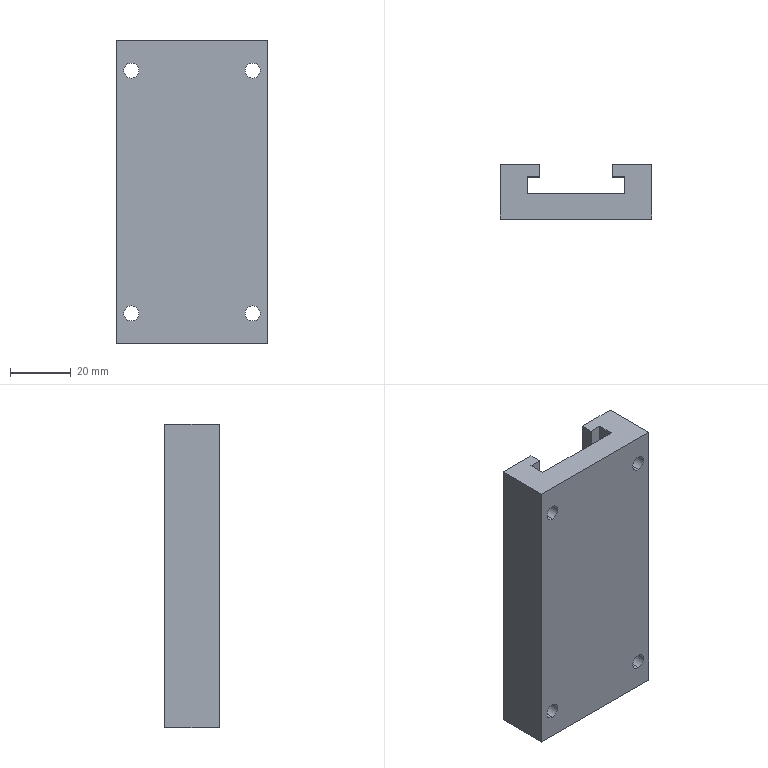Component | SolidWorks | 8TC-A15004-D0-13A-2 | 1 solid | 22 faces | box 50 x 18 x 100 mm | volume 61386 mm3 | plane 14 | cylinder 8 | commonest cylinder face diameters 5 x8 | material #45
build123d program:
from build123d import *

# Parameters (mm, degrees)
SKETCH1_W           = 100
SKETCH1_H           = 50
BOSS_EXTRUDE1_DEPTH = 18
CUT_EXTRUDE1_DEPTH  = 105.637
M6_TAPPED_HOLE1_D   = 5


with BuildPart() as part:
    # Sketch1 → Boss-Extrude1 (new body)
    with BuildSketch(Plane.XY):
        Rectangle(SKETCH1_W, SKETCH1_H)
    extrude(amount=BOSS_EXTRUDE1_DEPTH)

    # Sketch2 → Cut-Extrude1 (cut, through all)
    with BuildSketch(Plane(origin=(50, 0, 0), x_dir=(0, 0, -1), z_dir=(1, 0, 0))):
        Polygon((-8.5, -16), (-8.5, 16), (-14, 16), (-14, 12), (-18, 12), (-18, -12), (-14, -12), (-14, -16), align=None)
    extrude(amount=-CUT_EXTRUDE1_DEPTH, mode=Mode.SUBTRACT)

    # M6 Tapped Hole1 (through all)
    with Locations(Plane(origin=(0, 0, 0), x_dir=(-1, 0, 0), z_dir=(0, 0, -1))):
        with Locations((-40, 20), (-40, -20), (40, -20), (40, 20)):
            Hole(M6_TAPPED_HOLE1_D / 2)


solid = part.part

# Placed as in the assembly
solid = solid.moved(Location((-7.5, 344.5, 0), (-90, 0, 90)))
STEP:
#1=COLOUR_RGB('',0.7922,0.8196,0.9333);
#2=FILL_AREA_STYLE_COLOUR('',#1);
#3=FILL_AREA_STYLE('',(#2));
#4=SURFACE_STYLE_FILL_AREA(#3);
#5=SURFACE_SIDE_STYLE('',(#4));
#6=SURFACE_STYLE_USAGE(.BOTH.,#5);
#7=PRESENTATION_STYLE_ASSIGNMENT((#6));
#8=CARTESIAN_POINT('',(-1.083,14.272,-1.673));
#9=VERTEX_POINT('',#8);
#10=CARTESIAN_POINT('',(-1.083,14.272,-1.476));
#11=VERTEX_POINT('',#10);
#12=CARTESIAN_POINT('',(-1.083,14.272,-1.575));
#13=DIRECTION('',(0.,-1.,-0.));
#14=DIRECTION('',(0.,0.,1.));
#15=AXIS2_PLACEMENT_3D('',#12,#13,#14);
#16=CIRCLE('',#15,0.09843);
#17=EDGE_CURVE('',#9,#11,#16,.T.);
#18=ORIENTED_EDGE('',*,*,#17,.F.);
#19=CARTESIAN_POINT('',(-1.083,13.563,-1.673));
#20=VERTEX_POINT('',#19);
#21=CARTESIAN_POINT('',(-1.083,13.563,-1.673));
#22=DIRECTION('',(0.,-1.,-0.));
#23=VECTOR('',#22,39.37);
#24=LINE('',#21,#23);
#25=EDGE_CURVE('',#9,#20,#24,.T.);
#26=ORIENTED_EDGE('',*,*,#25,.T.);
#27=CARTESIAN_POINT('',(-1.083,13.563,-1.476));
#28=VERTEX_POINT('',#27);
#29=CARTESIAN_POINT('',(-1.083,13.563,-1.575));
#30=DIRECTION('',(0.,-1.,-0.));
#31=DIRECTION('',(0.,0.,1.));
#32=AXIS2_PLACEMENT_3D('',#29,#30,#31);
#33=CIRCLE('',#32,0.09843);
#34=EDGE_CURVE('',#20,#28,#33,.T.);
#35=ORIENTED_EDGE('',*,*,#34,.T.);
#36=CARTESIAN_POINT('',(-1.083,13.563,-1.476));
#37=DIRECTION('',(0.,-1.,-0.));
#38=VECTOR('',#37,39.37);
#39=LINE('',#36,#38);
#40=EDGE_CURVE('',#11,#28,#39,.T.);
#41=ORIENTED_EDGE('',*,*,#40,.F.);
#42=EDGE_LOOP('',(#18,#26,#35,#41));
#43=FACE_OUTER_BOUND('',#42,.T.);
#44=CARTESIAN_POINT('',(-1.083,13.563,-1.575));
#45=DIRECTION('',(0.,-1.,-0.));
#46=DIRECTION('',(0.,0.,1.));
#47=AXIS2_PLACEMENT_3D('',#44,#45,#46);
#48=CYLINDRICAL_SURFACE('',#47,0.09843);
#49=ADVANCED_FACE('',(#43),#48,.F.);
#50=CARTESIAN_POINT('',(0.4921,14.272,-1.673));
#51=VERTEX_POINT('',#50);
#52=CARTESIAN_POINT('',(0.4921,14.272,-1.476));
#53=VERTEX_POINT('',#52);
#54=CARTESIAN_POINT('',(0.4921,14.272,-1.575));
#55=DIRECTION('',(0.,-1.,-0.));
#56=DIRECTION('',(0.,0.,1.));
#57=AXIS2_PLACEMENT_3D('',#54,#55,#56);
#58=CIRCLE('',#57,0.09843);
#59=EDGE_CURVE('',#51,#53,#58,.T.);
#60=ORIENTED_EDGE('',*,*,#59,.F.);
#61=CARTESIAN_POINT('',(0.4921,13.563,-1.673));
#62=VERTEX_POINT('',#61);
#63=CARTESIAN_POINT('',(0.4921,13.563,-1.673));
#64=DIRECTION('',(0.,-1.,-0.));
#65=VECTOR('',#64,39.37);
#66=LINE('',#63,#65);
#67=EDGE_CURVE('',#51,#62,#66,.T.);
#68=ORIENTED_EDGE('',*,*,#67,.T.);
#69=CARTESIAN_POINT('',(0.4921,13.563,-1.476));
#70=VERTEX_POINT('',#69);
#71=CARTESIAN_POINT('',(0.4921,13.563,-1.575));
#72=DIRECTION('',(0.,-1.,-0.));
#73=DIRECTION('',(0.,0.,1.));
#74=AXIS2_PLACEMENT_3D('',#71,#72,#73);
#75=CIRCLE('',#74,0.09843);
#76=EDGE_CURVE('',#62,#70,#75,.T.);
#77=ORIENTED_EDGE('',*,*,#76,.T.);
#78=CARTESIAN_POINT('',(0.4921,13.563,-1.476));
#79=DIRECTION('',(0.,-1.,-0.));
#80=VECTOR('',#79,39.37);
#81=LINE('',#78,#80);
#82=EDGE_CURVE('',#53,#70,#81,.T.);
#83=ORIENTED_EDGE('',*,*,#82,.F.);
#84=EDGE_LOOP('',(#60,#68,#77,#83));
#85=FACE_OUTER_BOUND('',#84,.T.);
#86=CARTESIAN_POINT('',(0.4921,13.563,-1.575));
#87=DIRECTION('',(0.,-1.,-0.));
#88=DIRECTION('',(0.,0.,1.));
#89=AXIS2_PLACEMENT_3D('',#86,#87,#88);
#90=CYLINDRICAL_SURFACE('',#89,0.09843);
#91=ADVANCED_FACE('',(#85),#90,.F.);
#92=CARTESIAN_POINT('',(0.4921,14.272,1.476));
#93=VERTEX_POINT('',#92);
#94=CARTESIAN_POINT('',(0.4921,14.272,1.673));
#95=VERTEX_POINT('',#94);
#96=CARTESIAN_POINT('',(0.4921,14.272,1.575));
#97=DIRECTION('',(0.,-1.,-0.));
#98=DIRECTION('',(0.,0.,1.));
#99=AXIS2_PLACEMENT_3D('',#96,#97,#98);
#100=CIRCLE('',#99,0.09843);
#101=EDGE_CURVE('',#93,#95,#100,.T.);
#102=ORIENTED_EDGE('',*,*,#101,.F.);
#103=CARTESIAN_POINT('',(0.4921,13.563,1.476));
#104=VERTEX_POINT('',#103);
#105=CARTESIAN_POINT('',(0.4921,13.563,1.476));
#106=DIRECTION('',(0.,-1.,-0.));
#107=VECTOR('',#106,39.37);
#108=LINE('',#105,#107);
#109=EDGE_CURVE('',#93,#104,#108,.T.);
#110=ORIENTED_EDGE('',*,*,#109,.T.);
#111=CARTESIAN_POINT('',(0.4921,13.563,1.673));
#112=VERTEX_POINT('',#111);
#113=CARTESIAN_POINT('',(0.4921,13.563,1.575));
#114=DIRECTION('',(0.,-1.,-0.));
#115=DIRECTION('',(0.,0.,1.));
#116=AXIS2_PLACEMENT_3D('',#113,#114,#115);
#117=CIRCLE('',#116,0.09843);
#118=EDGE_CURVE('',#104,#112,#117,.T.);
#119=ORIENTED_EDGE('',*,*,#118,.T.);
#120=CARTESIAN_POINT('',(0.4921,13.563,1.673));
#121=DIRECTION('',(0.,-1.,-0.));
#122=VECTOR('',#121,39.37);
#123=LINE('',#120,#122);
#124=EDGE_CURVE('',#95,#112,#123,.T.);
#125=ORIENTED_EDGE('',*,*,#124,.F.);
#126=EDGE_LOOP('',(#102,#110,#119,#125));
#127=FACE_OUTER_BOUND('',#126,.T.);
#128=CARTESIAN_POINT('',(0.4921,13.563,1.575));
#129=DIRECTION('',(0.,-1.,-0.));
#130=DIRECTION('',(0.,0.,1.));
#131=AXIS2_PLACEMENT_3D('',#128,#129,#130);
#132=CYLINDRICAL_SURFACE('',#131,0.09843);
#133=ADVANCED_FACE('',(#127),#132,.F.);
#134=CARTESIAN_POINT('',(-1.083,14.272,1.476));
#135=VERTEX_POINT('',#134);
#136=CARTESIAN_POINT('',(-1.083,14.272,1.673));
#137=VERTEX_POINT('',#136);
#138=CARTESIAN_POINT('',(-1.083,14.272,1.575));
#139=DIRECTION('',(0.,-1.,-0.));
#140=DIRECTION('',(0.,0.,1.));
#141=AXIS2_PLACEMENT_3D('',#138,#139,#140);
#142=CIRCLE('',#141,0.09843);
#143=EDGE_CURVE('',#135,#137,#142,.T.);
#144=ORIENTED_EDGE('',*,*,#143,.F.);
#145=CARTESIAN_POINT('',(-1.083,13.563,1.476));
#146=VERTEX_POINT('',#145);
#147=CARTESIAN_POINT('',(-1.083,13.563,1.476));
#148=DIRECTION('',(0.,-1.,-0.));
#149=VECTOR('',#148,39.37);
#150=LINE('',#147,#149);
#151=EDGE_CURVE('',#135,#146,#150,.T.);
#152=ORIENTED_EDGE('',*,*,#151,.T.);
#153=CARTESIAN_POINT('',(-1.083,13.563,1.673));
#154=VERTEX_POINT('',#153);
#155=CARTESIAN_POINT('',(-1.083,13.563,1.575));
#156=DIRECTION('',(0.,-1.,-0.));
#157=DIRECTION('',(0.,0.,1.));
#158=AXIS2_PLACEMENT_3D('',#155,#156,#157);
#159=CIRCLE('',#158,0.09843);
#160=EDGE_CURVE('',#146,#154,#159,.T.);
#161=ORIENTED_EDGE('',*,*,#160,.T.);
#162=CARTESIAN_POINT('',(-1.083,13.563,1.673));
#163=DIRECTION('',(0.,-1.,-0.));
#164=VECTOR('',#163,39.37);
#165=LINE('',#162,#164);
#166=EDGE_CURVE('',#137,#154,#165,.T.);
#167=ORIENTED_EDGE('',*,*,#166,.F.);
#168=EDGE_LOOP('',(#144,#152,#161,#167));
#169=FACE_OUTER_BOUND('',#168,.T.);
#170=CARTESIAN_POINT('',(-1.083,13.563,1.575));
#171=DIRECTION('',(0.,-1.,-0.));
#172=DIRECTION('',(0.,0.,1.));
#173=AXIS2_PLACEMENT_3D('',#170,#171,#172);
#174=CYLINDRICAL_SURFACE('',#173,0.09843);
#175=ADVANCED_FACE('',(#169),#174,.F.);
#176=CARTESIAN_POINT('',(0.4921,14.272,-1.575));
#177=DIRECTION('',(0.,-1.,-0.));
#178=DIRECTION('',(0.,0.,1.));
#179=AXIS2_PLACEMENT_3D('',#176,#177,#178);
#180=CIRCLE('',#179,0.09843);
#181=EDGE_CURVE('',#53,#51,#180,.T.);
#182=ORIENTED_EDGE('',*,*,#181,.T.);
#183=ORIENTED_EDGE('',*,*,#59,.T.);
#184=EDGE_LOOP('',(#182,#183));
#185=FACE_BOUND('',#184,.T.);
#186=CARTESIAN_POINT('',(0.4921,14.272,1.575));
#187=DIRECTION('',(0.,-1.,-0.));
#188=DIRECTION('',(0.,0.,1.));
#189=AXIS2_PLACEMENT_3D('',#186,#187,#188);
#190=CIRCLE('',#189,0.09843);
#191=EDGE_CURVE('',#95,#93,#190,.T.);
#192=ORIENTED_EDGE('',*,*,#191,.T.);
#193=ORIENTED_EDGE('',*,*,#101,.T.);
#194=EDGE_LOOP('',(#192,#193));
#195=FACE_BOUND('',#194,.T.);
#196=CARTESIAN_POINT('',(0.689,14.272,-1.969));
#197=VERTEX_POINT('',#196);
#198=CARTESIAN_POINT('',(0.1772,14.272,-1.969));
#199=VERTEX_POINT('',#198);
#200=CARTESIAN_POINT('',(0.689,14.272,-1.969));
#201=DIRECTION('',(-1.,-0.,-0.));
#202=VECTOR('',#201,39.37);
#203=LINE('',#200,#202);
#204=EDGE_CURVE('',#197,#199,#203,.T.);
#205=ORIENTED_EDGE('',*,*,#204,.T.);
#206=CARTESIAN_POINT('',(0.1772,14.272,1.969));
#207=VERTEX_POINT('',#206);
#208=CARTESIAN_POINT('',(0.1772,14.272,1.969));
#209=DIRECTION('',(0.,0.,-1.));
#210=VECTOR('',#209,39.37);
#211=LINE('',#208,#210);
#212=EDGE_CURVE('',#207,#199,#211,.T.);
#213=ORIENTED_EDGE('',*,*,#212,.F.);
#214=CARTESIAN_POINT('',(0.689,14.272,1.969));
#215=VERTEX_POINT('',#214);
#216=CARTESIAN_POINT('',(0.689,14.272,1.969));
#217=DIRECTION('',(1.,0.,0.));
#218=VECTOR('',#217,39.37);
#219=LINE('',#216,#218);
#220=EDGE_CURVE('',#207,#215,#219,.T.);
#221=ORIENTED_EDGE('',*,*,#220,.T.);
#222=CARTESIAN_POINT('',(0.689,14.272,1.969));
#223=DIRECTION('',(0.,0.,-1.));
#224=VECTOR('',#223,39.37);
#225=LINE('',#222,#224);
#226=EDGE_CURVE('',#215,#197,#225,.T.);
#227=ORIENTED_EDGE('',*,*,#226,.T.);
#228=EDGE_LOOP('',(#205,#213,#221,#227));
#229=FACE_OUTER_BOUND('',#228,.T.);
#230=CARTESIAN_POINT('',(-0.2953,14.272,-0.));
#231=DIRECTION('',(0.,-1.,-0.));
#232=DIRECTION('',(-0.,-0.,1.));
#233=AXIS2_PLACEMENT_3D('',#230,#231,#232);
#234=PLANE('',#233);
#235=ADVANCED_FACE('',(#185,#195,#229),#234,.F.);
#236=CARTESIAN_POINT('',(0.1772,14.114,-1.969));
#237=VERTEX_POINT('',#236);
#238=CARTESIAN_POINT('',(0.3346,14.114,-1.969));
#239=VERTEX_POINT('',#238);
#240=CARTESIAN_POINT('',(0.3346,14.114,-1.969));
#241=DIRECTION('',(1.,0.,0.));
#242=VECTOR('',#241,39.37);
#243=LINE('',#240,#242);
#244=EDGE_CURVE('',#237,#239,#243,.T.);
#245=ORIENTED_EDGE('',*,*,#244,.F.);
#246=CARTESIAN_POINT('',(0.1772,14.114,-1.969));
#247=DIRECTION('',(0.,-1.,-0.));
#248=VECTOR('',#247,39.37);
#249=LINE('',#246,#248);
#250=EDGE_CURVE('',#199,#237,#249,.T.);
#251=ORIENTED_EDGE('',*,*,#250,.F.);
#252=ORIENTED_EDGE('',*,*,#204,.F.);
#253=CARTESIAN_POINT('',(0.689,13.563,-1.969));
#254=VERTEX_POINT('',#253);
#255=CARTESIAN_POINT('',(0.689,14.272,-1.969));
#256=DIRECTION('',(0.,-1.,-0.));
#257=VECTOR('',#256,39.37);
#258=LINE('',#255,#257);
#259=EDGE_CURVE('',#197,#254,#258,.T.);
#260=ORIENTED_EDGE('',*,*,#259,.T.);
#261=CARTESIAN_POINT('',(-1.28,13.563,-1.969));
#262=VERTEX_POINT('',#261);
#263=CARTESIAN_POINT('',(0.689,13.563,-1.969));
#264=DIRECTION('',(-1.,-0.,-0.));
#265=VECTOR('',#264,39.37);
#266=LINE('',#263,#265);
#267=EDGE_CURVE('',#254,#262,#266,.T.);
#268=ORIENTED_EDGE('',*,*,#267,.T.);
#269=CARTESIAN_POINT('',(-1.28,14.272,-1.969));
#270=VERTEX_POINT('',#269);
#271=CARTESIAN_POINT('',(-1.28,14.272,-1.969));
#272=DIRECTION('',(0.,-1.,-0.));
#273=VECTOR('',#272,39.37);
#274=LINE('',#271,#273);
#275=EDGE_CURVE('',#270,#262,#274,.T.);
#276=ORIENTED_EDGE('',*,*,#275,.F.);
#277=CARTESIAN_POINT('',(-0.7677,14.272,-1.969));
#278=VERTEX_POINT('',#277);
#279=CARTESIAN_POINT('',(0.689,14.272,-1.969));
#280=DIRECTION('',(-1.,-0.,-0.));
#281=VECTOR('',#280,39.37);
#282=LINE('',#279,#281);
#283=EDGE_CURVE('',#278,#270,#282,.T.);
#284=ORIENTED_EDGE('',*,*,#283,.F.);
#285=CARTESIAN_POINT('',(-0.7677,14.114,-1.969));
#286=VERTEX_POINT('',#285);
#287=CARTESIAN_POINT('',(-0.7677,14.114,-1.969));
#288=DIRECTION('',(0.,1.,0.));
#289=VECTOR('',#288,39.37);
#290=LINE('',#287,#289);
#291=EDGE_CURVE('',#286,#278,#290,.T.);
#292=ORIENTED_EDGE('',*,*,#291,.F.);
#293=CARTESIAN_POINT('',(-0.9252,14.114,-1.969));
#294=VERTEX_POINT('',#293);
#295=CARTESIAN_POINT('',(-0.9252,14.114,-1.969));
#296=DIRECTION('',(1.,0.,0.));
#297=VECTOR('',#296,39.37);
#298=LINE('',#295,#297);
#299=EDGE_CURVE('',#294,#286,#298,.T.);
#300=ORIENTED_EDGE('',*,*,#299,.F.);
#301=CARTESIAN_POINT('',(-0.9252,13.898,-1.969));
#302=VERTEX_POINT('',#301);
#303=CARTESIAN_POINT('',(-0.9252,13.898,-1.969));
#304=DIRECTION('',(-0.,1.,0.));
#305=VECTOR('',#304,39.37);
#306=LINE('',#303,#305);
#307=EDGE_CURVE('',#302,#294,#306,.T.);
#308=ORIENTED_EDGE('',*,*,#307,.F.);
#309=CARTESIAN_POINT('',(0.3346,13.898,-1.969));
#310=VERTEX_POINT('',#309);
#311=CARTESIAN_POINT('',(0.3346,13.898,-1.969));
#312=DIRECTION('',(-1.,-0.,-0.));
#313=VECTOR('',#312,39.37);
#314=LINE('',#311,#313);
#315=EDGE_CURVE('',#310,#302,#314,.T.);
#316=ORIENTED_EDGE('',*,*,#315,.F.);
#317=CARTESIAN_POINT('',(0.3346,13.898,-1.969));
#318=DIRECTION('',(0.,-1.,-0.));
#319=VECTOR('',#318,39.37);
#320=LINE('',#317,#319);
#321=EDGE_CURVE('',#239,#310,#320,.T.);
#322=ORIENTED_EDGE('',*,*,#321,.F.);
#323=EDGE_LOOP('',(#245,#251,#252,#260,#268,#276,#284,#292,#300,#308,#316,#322));
#324=FACE_OUTER_BOUND('',#323,.T.);
#325=CARTESIAN_POINT('',(0.689,14.272,-1.969));
#326=DIRECTION('',(-0.,-0.,1.));
#327=DIRECTION('',(-0.,1.,0.));
#328=AXIS2_PLACEMENT_3D('',#325,#326,#327);
#329=PLANE('',#328);
#330=ADVANCED_FACE('',(#324),#329,.F.);
#331=CARTESIAN_POINT('',(-1.28,13.563,1.969));
#332=VERTEX_POINT('',#331);
#333=CARTESIAN_POINT('',(-1.28,13.563,1.969));
#334=DIRECTION('',(-0.,-0.,1.));
#335=VECTOR('',#334,39.37);
#336=LINE('',#333,#335);
#337=EDGE_CURVE('',#262,#332,#336,.T.);
#338=ORIENTED_EDGE('',*,*,#337,.T.);
#339=CARTESIAN_POINT('',(-1.28,14.272,1.969));
#340=VERTEX_POINT('',#339);
#341=CARTESIAN_POINT('',(-1.28,14.272,1.969));
#342=DIRECTION('',(0.,-1.,-0.));
#343=VECTOR('',#342,39.37);
#344=LINE('',#341,#343);
#345=EDGE_CURVE('',#340,#332,#344,.T.);
#346=ORIENTED_EDGE('',*,*,#345,.F.);
#347=CARTESIAN_POINT('',(-1.28,14.272,1.969));
#348=DIRECTION('',(-0.,-0.,1.));
#349=VECTOR('',#348,39.37);
#350=LINE('',#347,#349);
#351=EDGE_CURVE('',#270,#340,#350,.T.);
#352=ORIENTED_EDGE('',*,*,#351,.F.);
#353=ORIENTED_EDGE('',*,*,#275,.T.);
#354=EDGE_LOOP('',(#338,#346,#352,#353));
#355=FACE_OUTER_BOUND('',#354,.T.);
#356=CARTESIAN_POINT('',(-1.28,14.272,1.969));
#357=DIRECTION('',(1.,0.,0.));
#358=DIRECTION('',(0.,-1.,-0.));
#359=AXIS2_PLACEMENT_3D('',#356,#357,#358);
#360=PLANE('',#359);
#361=ADVANCED_FACE('',(#355),#360,.F.);
#362=ORIENTED_EDGE('',*,*,#220,.F.);
#363=CARTESIAN_POINT('',(0.1772,14.114,1.969));
#364=VERTEX_POINT('',#363);
#365=CARTESIAN_POINT('',(0.1772,14.114,1.969));
#366=DIRECTION('',(0.,-1.,-0.));
#367=VECTOR('',#366,39.37);
#368=LINE('',#365,#367);
#369=EDGE_CURVE('',#207,#364,#368,.T.);
#370=ORIENTED_EDGE('',*,*,#369,.T.);
#371=CARTESIAN_POINT('',(0.3346,14.114,1.969));
#372=VERTEX_POINT('',#371);
#373=CARTESIAN_POINT('',(0.3346,14.114,1.969));
#374=DIRECTION('',(1.,0.,0.));
#375=VECTOR('',#374,39.37);
#376=LINE('',#373,#375);
#377=EDGE_CURVE('',#364,#372,#376,.T.);
#378=ORIENTED_EDGE('',*,*,#377,.T.);
#379=CARTESIAN_POINT('',(0.3346,13.898,1.969));
#380=VERTEX_POINT('',#379);
#381=CARTESIAN_POINT('',(0.3346,13.898,1.969));
#382=DIRECTION('',(0.,-1.,-0.));
#383=VECTOR('',#382,39.37);
#384=LINE('',#381,#383);
#385=EDGE_CURVE('',#372,#380,#384,.T.);
#386=ORIENTED_EDGE('',*,*,#385,.T.);
#387=CARTESIAN_POINT('',(-0.9252,13.898,1.969));
#388=VERTEX_POINT('',#387);
#389=CARTESIAN_POINT('',(0.3346,13.898,1.969));
#390=DIRECTION('',(-1.,-0.,-0.));
#391=VECTOR('',#390,39.37);
#392=LINE('',#389,#391);
#393=EDGE_CURVE('',#380,#388,#392,.T.);
#394=ORIENTED_EDGE('',*,*,#393,.T.);
#395=CARTESIAN_POINT('',(-0.9252,14.114,1.969));
#396=VERTEX_POINT('',#395);
#397=CARTESIAN_POINT('',(-0.9252,13.898,1.969));
#398=DIRECTION('',(-0.,1.,0.));
#399=VECTOR('',#398,39.37);
#400=LINE('',#397,#399);
#401=EDGE_CURVE('',#388,#396,#400,.T.);
#402=ORIENTED_EDGE('',*,*,#401,.T.);
#403=CARTESIAN_POINT('',(-0.7677,14.114,1.969));
#404=VERTEX_POINT('',#403);
#405=CARTESIAN_POINT('',(-0.9252,14.114,1.969));
#406=DIRECTION('',(1.,0.,0.));
#407=VECTOR('',#406,39.37);
#408=LINE('',#405,#407);
#409=EDGE_CURVE('',#396,#404,#408,.T.);
#410=ORIENTED_EDGE('',*,*,#409,.T.);
#411=CARTESIAN_POINT('',(-0.7677,14.272,1.969));
#412=VERTEX_POINT('',#411);
#413=CARTESIAN_POINT('',(-0.7677,14.114,1.969));
#414=DIRECTION('',(0.,1.,0.));
#415=VECTOR('',#414,39.37);
#416=LINE('',#413,#415);
#417=EDGE_CURVE('',#404,#412,#416,.T.);
#418=ORIENTED_EDGE('',*,*,#417,.T.);
#419=CARTESIAN_POINT('',(0.689,14.272,1.969));
#420=DIRECTION('',(1.,0.,0.));
#421=VECTOR('',#420,39.37);
#422=LINE('',#419,#421);
#423=EDGE_CURVE('',#340,#412,#422,.T.);
#424=ORIENTED_EDGE('',*,*,#423,.F.);
#425=ORIENTED_EDGE('',*,*,#345,.T.);
#426=CARTESIAN_POINT('',(0.689,13.563,1.969));
#427=VERTEX_POINT('',#426);
#428=CARTESIAN_POINT('',(0.689,13.563,1.969));
#429=DIRECTION('',(1.,0.,0.));
#430=VECTOR('',#429,39.37);
#431=LINE('',#428,#430);
#432=EDGE_CURVE('',#332,#427,#431,.T.);
#433=ORIENTED_EDGE('',*,*,#432,.T.);
#434=CARTESIAN_POINT('',(0.689,14.272,1.969));
#435=DIRECTION('',(0.,-1.,-0.));
#436=VECTOR('',#435,39.37);
#437=LINE('',#434,#436);
#438=EDGE_CURVE('',#215,#427,#437,.T.);
#439=ORIENTED_EDGE('',*,*,#438,.F.);
#440=EDGE_LOOP('',(#362,#370,#378,#386,#394,#402,#410,#418,#424,#425,#433,#439));
#441=FACE_OUTER_BOUND('',#440,.T.);
#442=CARTESIAN_POINT('',(0.689,14.272,1.969));
#443=DIRECTION('',(0.,0.,-1.));
#444=DIRECTION('',(0.,-1.,-0.));
#445=AXIS2_PLACEMENT_3D('',#442,#443,#444);
#446=PLANE('',#445);
#447=ADVANCED_FACE('',(#441),#446,.F.);
#448=CARTESIAN_POINT('',(0.689,13.563,1.969));
#449=DIRECTION('',(0.,0.,-1.));
#450=VECTOR('',#449,39.37);
#451=LINE('',#448,#450);
#452=EDGE_CURVE('',#427,#254,#451,.T.);
#453=ORIENTED_EDGE('',*,*,#452,.T.);
#454=ORIENTED_EDGE('',*,*,#259,.F.);
#455=ORIENTED_EDGE('',*,*,#226,.F.);
#456=ORIENTED_EDGE('',*,*,#438,.T.);
#457=EDGE_LOOP('',(#453,#454,#455,#456));
#458=FACE_OUTER_BOUND('',#457,.T.);
#459=CARTESIAN_POINT('',(0.689,14.272,1.969));
#460=DIRECTION('',(-1.,-0.,-0.));
#461=DIRECTION('',(-0.,1.,0.));
#462=AXIS2_PLACEMENT_3D('',#459,#460,#461);
#463=PLANE('',#462);
#464=ADVANCED_FACE('',(#458),#463,.F.);
#465=CARTESIAN_POINT('',(-1.083,14.272,-1.575));
#466=DIRECTION('',(0.,-1.,-0.));
#467=DIRECTION('',(0.,0.,1.));
#468=AXIS2_PLACEMENT_3D('',#465,#466,#467);
#469=CIRCLE('',#468,0.09843);
#470=EDGE_CURVE('',#11,#9,#469,.T.);
#471=ORIENTED_EDGE('',*,*,#470,.T.);
#472=ORIENTED_EDGE('',*,*,#17,.T.);
#473=EDGE_LOOP('',(#471,#472));
#474=FACE_BOUND('',#473,.T.);
#475=CARTESIAN_POINT('',(-1.083,14.272,1.575));
#476=DIRECTION('',(0.,-1.,-0.));
#477=DIRECTION('',(0.,0.,1.));
#478=AXIS2_PLACEMENT_3D('',#475,#476,#477);
#479=CIRCLE('',#478,0.09843);
#480=EDGE_CURVE('',#137,#135,#479,.T.);
#481=ORIENTED_EDGE('',*,*,#480,.T.);
#482=ORIENTED_EDGE('',*,*,#143,.T.);
#483=EDGE_LOOP('',(#481,#482));
#484=FACE_BOUND('',#483,.T.);
#485=ORIENTED_EDGE('',*,*,#423,.T.);
#486=CARTESIAN_POINT('',(-0.7677,14.272,1.969));
#487=DIRECTION('',(0.,0.,-1.));
#488=VECTOR('',#487,39.37);
#489=LINE('',#486,#488);
#490=EDGE_CURVE('',#412,#278,#489,.T.);
#491=ORIENTED_EDGE('',*,*,#490,.T.);
#492=ORIENTED_EDGE('',*,*,#283,.T.);
#493=ORIENTED_EDGE('',*,*,#351,.T.);
#494=EDGE_LOOP('',(#485,#491,#492,#493));
#495=FACE_OUTER_BOUND('',#494,.T.);
#496=CARTESIAN_POINT('',(-0.2953,14.272,-0.));
#497=DIRECTION('',(0.,-1.,-0.));
#498=DIRECTION('',(-0.,-0.,1.));
#499=AXIS2_PLACEMENT_3D('',#496,#497,#498);
#500=PLANE('',#499);
#501=ADVANCED_FACE('',(#474,#484,#495),#500,.F.);
#502=CARTESIAN_POINT('',(-1.083,13.563,-1.575));
#503=DIRECTION('',(0.,-1.,-0.));
#504=DIRECTION('',(0.,0.,1.));
#505=AXIS2_PLACEMENT_3D('',#502,#503,#504);
#506=CIRCLE('',#505,0.09843);
#507=EDGE_CURVE('',#28,#20,#506,.T.);
#508=ORIENTED_EDGE('',*,*,#507,.F.);
#509=ORIENTED_EDGE('',*,*,#34,.F.);
#510=EDGE_LOOP('',(#508,#509));
#511=FACE_BOUND('',#510,.T.);
#512=CARTESIAN_POINT('',(0.4921,13.563,-1.575));
#513=DIRECTION('',(0.,-1.,-0.));
#514=DIRECTION('',(0.,0.,1.));
#515=AXIS2_PLACEMENT_3D('',#512,#513,#514);
#516=CIRCLE('',#515,0.09843);
#517=EDGE_CURVE('',#70,#62,#516,.T.);
#518=ORIENTED_EDGE('',*,*,#517,.F.);
#519=ORIENTED_EDGE('',*,*,#76,.F.);
#520=EDGE_LOOP('',(#518,#519));
#521=FACE_BOUND('',#520,.T.);
#522=CARTESIAN_POINT('',(0.4921,13.563,1.575));
#523=DIRECTION('',(0.,-1.,-0.));
#524=DIRECTION('',(0.,0.,1.));
#525=AXIS2_PLACEMENT_3D('',#522,#523,#524);
#526=CIRCLE('',#525,0.09843);
#527=EDGE_CURVE('',#112,#104,#526,.T.);
#528=ORIENTED_EDGE('',*,*,#527,.F.);
#529=ORIENTED_EDGE('',*,*,#118,.F.);
#530=EDGE_LOOP('',(#528,#529));
#531=FACE_BOUND('',#530,.T.);
#532=CARTESIAN_POINT('',(-1.083,13.563,1.575));
#533=DIRECTION('',(0.,-1.,-0.));
#534=DIRECTION('',(0.,0.,1.));
#535=AXIS2_PLACEMENT_3D('',#532,#533,#534);
#536=CIRCLE('',#535,0.09843);
#537=EDGE_CURVE('',#154,#146,#536,.T.);
#538=ORIENTED_EDGE('',*,*,#537,.F.);
#539=ORIENTED_EDGE('',*,*,#160,.F.);
#540=EDGE_LOOP('',(#538,#539));
#541=FACE_BOUND('',#540,.T.);
#542=ORIENTED_EDGE('',*,*,#267,.F.);
#543=ORIENTED_EDGE('',*,*,#452,.F.);
#544=ORIENTED_EDGE('',*,*,#432,.F.);
#545=ORIENTED_EDGE('',*,*,#337,.F.);
#546=EDGE_LOOP('',(#542,#543,#544,#545));
#547=FACE_OUTER_BOUND('',#546,.T.);
#548=CARTESIAN_POINT('',(-0.2953,13.563,-0.));
#549=DIRECTION('',(0.,-1.,-0.));
#550=DIRECTION('',(-0.,-0.,1.));
#551=AXIS2_PLACEMENT_3D('',#548,#549,#550);
#552=PLANE('',#551);
#553=ADVANCED_FACE('',(#511,#521,#531,#541,#547),#552,.T.);
#554=ORIENTED_EDGE('',*,*,#307,.T.);
#555=CARTESIAN_POINT('',(-0.9252,14.114,1.969));
#556=DIRECTION('',(0.,0.,-1.));
#557=VECTOR('',#556,39.37);
#558=LINE('',#555,#557);
#559=EDGE_CURVE('',#396,#294,#558,.T.);
#560=ORIENTED_EDGE('',*,*,#559,.F.);
#561=ORIENTED_EDGE('',*,*,#401,.F.);
#562=CARTESIAN_POINT('',(-0.9252,13.898,1.969));
#563=DIRECTION('',(0.,0.,-1.));
#564=VECTOR('',#563,39.37);
#565=LINE('',#562,#564);
#566=EDGE_CURVE('',#388,#302,#565,.T.);
#567=ORIENTED_EDGE('',*,*,#566,.T.);
#568=EDGE_LOOP('',(#554,#560,#561,#567));
#569=FACE_OUTER_BOUND('',#568,.T.);
#570=CARTESIAN_POINT('',(-0.9252,13.898,1.969));
#571=DIRECTION('',(-1.,-0.,-0.));
#572=DIRECTION('',(-0.,1.,0.));
#573=AXIS2_PLACEMENT_3D('',#570,#571,#572);
#574=PLANE('',#573);
#575=ADVANCED_FACE('',(#569),#574,.F.);
#576=ORIENTED_EDGE('',*,*,#315,.T.);
#577=ORIENTED_EDGE('',*,*,#566,.F.);
#578=ORIENTED_EDGE('',*,*,#393,.F.);
#579=CARTESIAN_POINT('',(0.3346,13.898,1.969));
#580=DIRECTION('',(0.,0.,-1.));
#581=VECTOR('',#580,39.37);
#582=LINE('',#579,#581);
#583=EDGE_CURVE('',#380,#310,#582,.T.);
#584=ORIENTED_EDGE('',*,*,#583,.T.);
#585=EDGE_LOOP('',(#576,#577,#578,#584));
#586=FACE_OUTER_BOUND('',#585,.T.);
#587=CARTESIAN_POINT('',(0.3346,13.898,1.969));
#588=DIRECTION('',(0.,-1.,-0.));
#589=DIRECTION('',(-1.,-0.,-0.));
#590=AXIS2_PLACEMENT_3D('',#587,#588,#589);
#591=PLANE('',#590);
#592=ADVANCED_FACE('',(#586),#591,.F.);
#593=ORIENTED_EDGE('',*,*,#321,.T.);
#594=ORIENTED_EDGE('',*,*,#583,.F.);
#595=ORIENTED_EDGE('',*,*,#385,.F.);
#596=CARTESIAN_POINT('',(0.3346,14.114,1.969));
#597=DIRECTION('',(0.,0.,-1.));
#598=VECTOR('',#597,39.37);
#599=LINE('',#596,#598);
#600=EDGE_CURVE('',#372,#239,#599,.T.);
#601=ORIENTED_EDGE('',*,*,#600,.T.);
#602=EDGE_LOOP('',(#593,#594,#595,#601));
#603=FACE_OUTER_BOUND('',#602,.T.);
#604=CARTESIAN_POINT('',(0.3346,13.898,1.969));
#605=DIRECTION('',(1.,0.,0.));
#606=DIRECTION('',(0.,-1.,-0.));
#607=AXIS2_PLACEMENT_3D('',#604,#605,#606);
#608=PLANE('',#607);
#609=ADVANCED_FACE('',(#603),#608,.F.);
#610=ORIENTED_EDGE('',*,*,#244,.T.);
#611=ORIENTED_EDGE('',*,*,#600,.F.);
#612=ORIENTED_EDGE('',*,*,#377,.F.);
#613=CARTESIAN_POINT('',(0.1772,14.114,1.969));
#614=DIRECTION('',(0.,0.,-1.));
#615=VECTOR('',#614,39.37);
#616=LINE('',#613,#615);
#617=EDGE_CURVE('',#364,#237,#616,.T.);
#618=ORIENTED_EDGE('',*,*,#617,.T.);
#619=EDGE_LOOP('',(#610,#611,#612,#618));
#620=FACE_OUTER_BOUND('',#619,.T.);
#621=CARTESIAN_POINT('',(0.3346,14.114,1.969));
#622=DIRECTION('',(-0.,1.,0.));
#623=DIRECTION('',(0.,0.,-1.));
#624=AXIS2_PLACEMENT_3D('',#621,#622,#623);
#625=PLANE('',#624);
#626=ADVANCED_FACE('',(#620),#625,.F.);
#627=ORIENTED_EDGE('',*,*,#250,.T.);
#628=ORIENTED_EDGE('',*,*,#617,.F.);
#629=ORIENTED_EDGE('',*,*,#369,.F.);
#630=ORIENTED_EDGE('',*,*,#212,.T.);
#631=EDGE_LOOP('',(#627,#628,#629,#630));
#632=FACE_OUTER_BOUND('',#631,.T.);
#633=CARTESIAN_POINT('',(0.1772,14.114,1.969));
#634=DIRECTION('',(1.,0.,0.));
#635=DIRECTION('',(0.,-1.,-0.));
#636=AXIS2_PLACEMENT_3D('',#633,#634,#635);
#637=PLANE('',#636);
#638=ADVANCED_FACE('',(#632),#637,.F.);
#639=ORIENTED_EDGE('',*,*,#291,.T.);
#640=ORIENTED_EDGE('',*,*,#490,.F.);
#641=ORIENTED_EDGE('',*,*,#417,.F.);
#642=CARTESIAN_POINT('',(-0.7677,14.114,1.969));
#643=DIRECTION('',(0.,0.,-1.));
#644=VECTOR('',#643,39.37);
#645=LINE('',#642,#644);
#646=EDGE_CURVE('',#404,#286,#645,.T.);
#647=ORIENTED_EDGE('',*,*,#646,.T.);
#648=EDGE_LOOP('',(#639,#640,#641,#647));
#649=FACE_OUTER_BOUND('',#648,.T.);
#650=CARTESIAN_POINT('',(-0.7677,14.114,1.969));
#651=DIRECTION('',(-1.,0.,-0.));
#652=DIRECTION('',(0.,1.,0.));
#653=AXIS2_PLACEMENT_3D('',#650,#651,#652);
#654=PLANE('',#653);
#655=ADVANCED_FACE('',(#649),#654,.F.);
#656=ORIENTED_EDGE('',*,*,#299,.T.);
#657=ORIENTED_EDGE('',*,*,#646,.F.);
#658=ORIENTED_EDGE('',*,*,#409,.F.);
#659=ORIENTED_EDGE('',*,*,#559,.T.);
#660=EDGE_LOOP('',(#656,#657,#658,#659));
#661=FACE_OUTER_BOUND('',#660,.T.);
#662=CARTESIAN_POINT('',(-0.9252,14.114,1.969));
#663=DIRECTION('',(-0.,1.,0.));
#664=DIRECTION('',(0.,0.,-1.));
#665=AXIS2_PLACEMENT_3D('',#662,#663,#664);
#666=PLANE('',#665);
#667=ADVANCED_FACE('',(#661),#666,.F.);
#668=ORIENTED_EDGE('',*,*,#151,.F.);
#669=ORIENTED_EDGE('',*,*,#480,.F.);
#670=ORIENTED_EDGE('',*,*,#166,.T.);
#671=ORIENTED_EDGE('',*,*,#537,.T.);
#672=EDGE_LOOP('',(#668,#669,#670,#671));
#673=FACE_OUTER_BOUND('',#672,.T.);
#674=CARTESIAN_POINT('',(-1.083,13.563,1.575));
#675=DIRECTION('',(0.,-1.,-0.));
#676=DIRECTION('',(0.,0.,1.));
#677=AXIS2_PLACEMENT_3D('',#674,#675,#676);
#678=CYLINDRICAL_SURFACE('',#677,0.09843);
#679=ADVANCED_FACE('',(#673),#678,.F.);
#680=ORIENTED_EDGE('',*,*,#109,.F.);
#681=ORIENTED_EDGE('',*,*,#191,.F.);
#682=ORIENTED_EDGE('',*,*,#124,.T.);
#683=ORIENTED_EDGE('',*,*,#527,.T.);
#684=EDGE_LOOP('',(#680,#681,#682,#683));
#685=FACE_OUTER_BOUND('',#684,.T.);
#686=CARTESIAN_POINT('',(0.4921,13.563,1.575));
#687=DIRECTION('',(0.,-1.,-0.));
#688=DIRECTION('',(0.,0.,1.));
#689=AXIS2_PLACEMENT_3D('',#686,#687,#688);
#690=CYLINDRICAL_SURFACE('',#689,0.09843);
#691=ADVANCED_FACE('',(#685),#690,.F.);
#692=ORIENTED_EDGE('',*,*,#67,.F.);
#693=ORIENTED_EDGE('',*,*,#181,.F.);
#694=ORIENTED_EDGE('',*,*,#82,.T.);
#695=ORIENTED_EDGE('',*,*,#517,.T.);
#696=EDGE_LOOP('',(#692,#693,#694,#695));
#697=FACE_OUTER_BOUND('',#696,.T.);
#698=CARTESIAN_POINT('',(0.4921,13.563,-1.575));
#699=DIRECTION('',(0.,-1.,-0.));
#700=DIRECTION('',(0.,0.,1.));
#701=AXIS2_PLACEMENT_3D('',#698,#699,#700);
#702=CYLINDRICAL_SURFACE('',#701,0.09843);
#703=ADVANCED_FACE('',(#697),#702,.F.);
#704=ORIENTED_EDGE('',*,*,#25,.F.);
#705=ORIENTED_EDGE('',*,*,#470,.F.);
#706=ORIENTED_EDGE('',*,*,#40,.T.);
#707=ORIENTED_EDGE('',*,*,#507,.T.);
#708=EDGE_LOOP('',(#704,#705,#706,#707));
#709=FACE_OUTER_BOUND('',#708,.T.);
#710=CARTESIAN_POINT('',(-1.083,13.563,-1.575));
#711=DIRECTION('',(0.,-1.,-0.));
#712=DIRECTION('',(0.,0.,1.));
#713=AXIS2_PLACEMENT_3D('',#710,#711,#712);
#714=CYLINDRICAL_SURFACE('',#713,0.09843);
#715=ADVANCED_FACE('',(#709),#714,.F.);
#716=CLOSED_SHELL('',(#49,#91,#133,#175,#235,#330,#361,#447,#464,#501,#553,#575,#592,#609,#626,#638,#655,#667,#679,#691,#703,#715));
#717=MANIFOLD_SOLID_BREP('',#716);
#718=STYLED_ITEM('',(#7),#717);
#719=PRESENTATION_LAYER_ASSIGNMENT('','',(#718));
#720=(LENGTH_UNIT()NAMED_UNIT(*)SI_UNIT($,.METRE.));
#721=LENGTH_MEASURE_WITH_UNIT(LENGTH_MEASURE(0.0254),#720);
#722=DIMENSIONAL_EXPONENTS(1.,0.,0.,0.,0.,0.,0.);
#723=(CONVERSION_BASED_UNIT('',#721)LENGTH_UNIT()NAMED_UNIT(#722));
#724=UNCERTAINTY_MEASURE_WITH_UNIT(LENGTH_MEASURE(0.00001),#723,'','');
#725=(NAMED_UNIT(*)PLANE_ANGLE_UNIT()SI_UNIT($,.RADIAN.));
#726=(NAMED_UNIT(*)SI_UNIT($,.STERADIAN.)SOLID_ANGLE_UNIT());
#727=(GEOMETRIC_REPRESENTATION_CONTEXT(3)GLOBAL_UNCERTAINTY_ASSIGNED_CONTEXT((#724))GLOBAL_UNIT_ASSIGNED_CONTEXT((#723,#725,#726))REPRESENTATION_CONTEXT('',''));
#728=MECHANICAL_DESIGN_GEOMETRIC_PRESENTATION_REPRESENTATION('',(#718),#727);
#729=CARTESIAN_POINT('',(0.,0.,0.));
#730=DIRECTION('',(0.,0.,1.));
#731=DIRECTION('',(1.,0.,0.));
#732=AXIS2_PLACEMENT_3D('',#729,#730,#731);
#733=(LENGTH_UNIT()NAMED_UNIT(*)SI_UNIT($,.METRE.));
#734=LENGTH_MEASURE_WITH_UNIT(LENGTH_MEASURE(0.0254),#733);
#735=DIMENSIONAL_EXPONENTS(1.,0.,0.,0.,0.,0.,0.);
#736=(CONVERSION_BASED_UNIT('',#734)LENGTH_UNIT()NAMED_UNIT(#735));
#737=UNCERTAINTY_MEASURE_WITH_UNIT(LENGTH_MEASURE(0.00001),#736,'','');
#738=(NAMED_UNIT(*)PLANE_ANGLE_UNIT()SI_UNIT($,.RADIAN.));
#739=(NAMED_UNIT(*)SI_UNIT($,.STERADIAN.)SOLID_ANGLE_UNIT());
#740=(GEOMETRIC_REPRESENTATION_CONTEXT(3)GLOBAL_UNCERTAINTY_ASSIGNED_CONTEXT((#737))GLOBAL_UNIT_ASSIGNED_CONTEXT((#736,#738,#739))REPRESENTATION_CONTEXT('',''));
#741=ADVANCED_BREP_SHAPE_REPRESENTATION('',(#717,#732),#740);